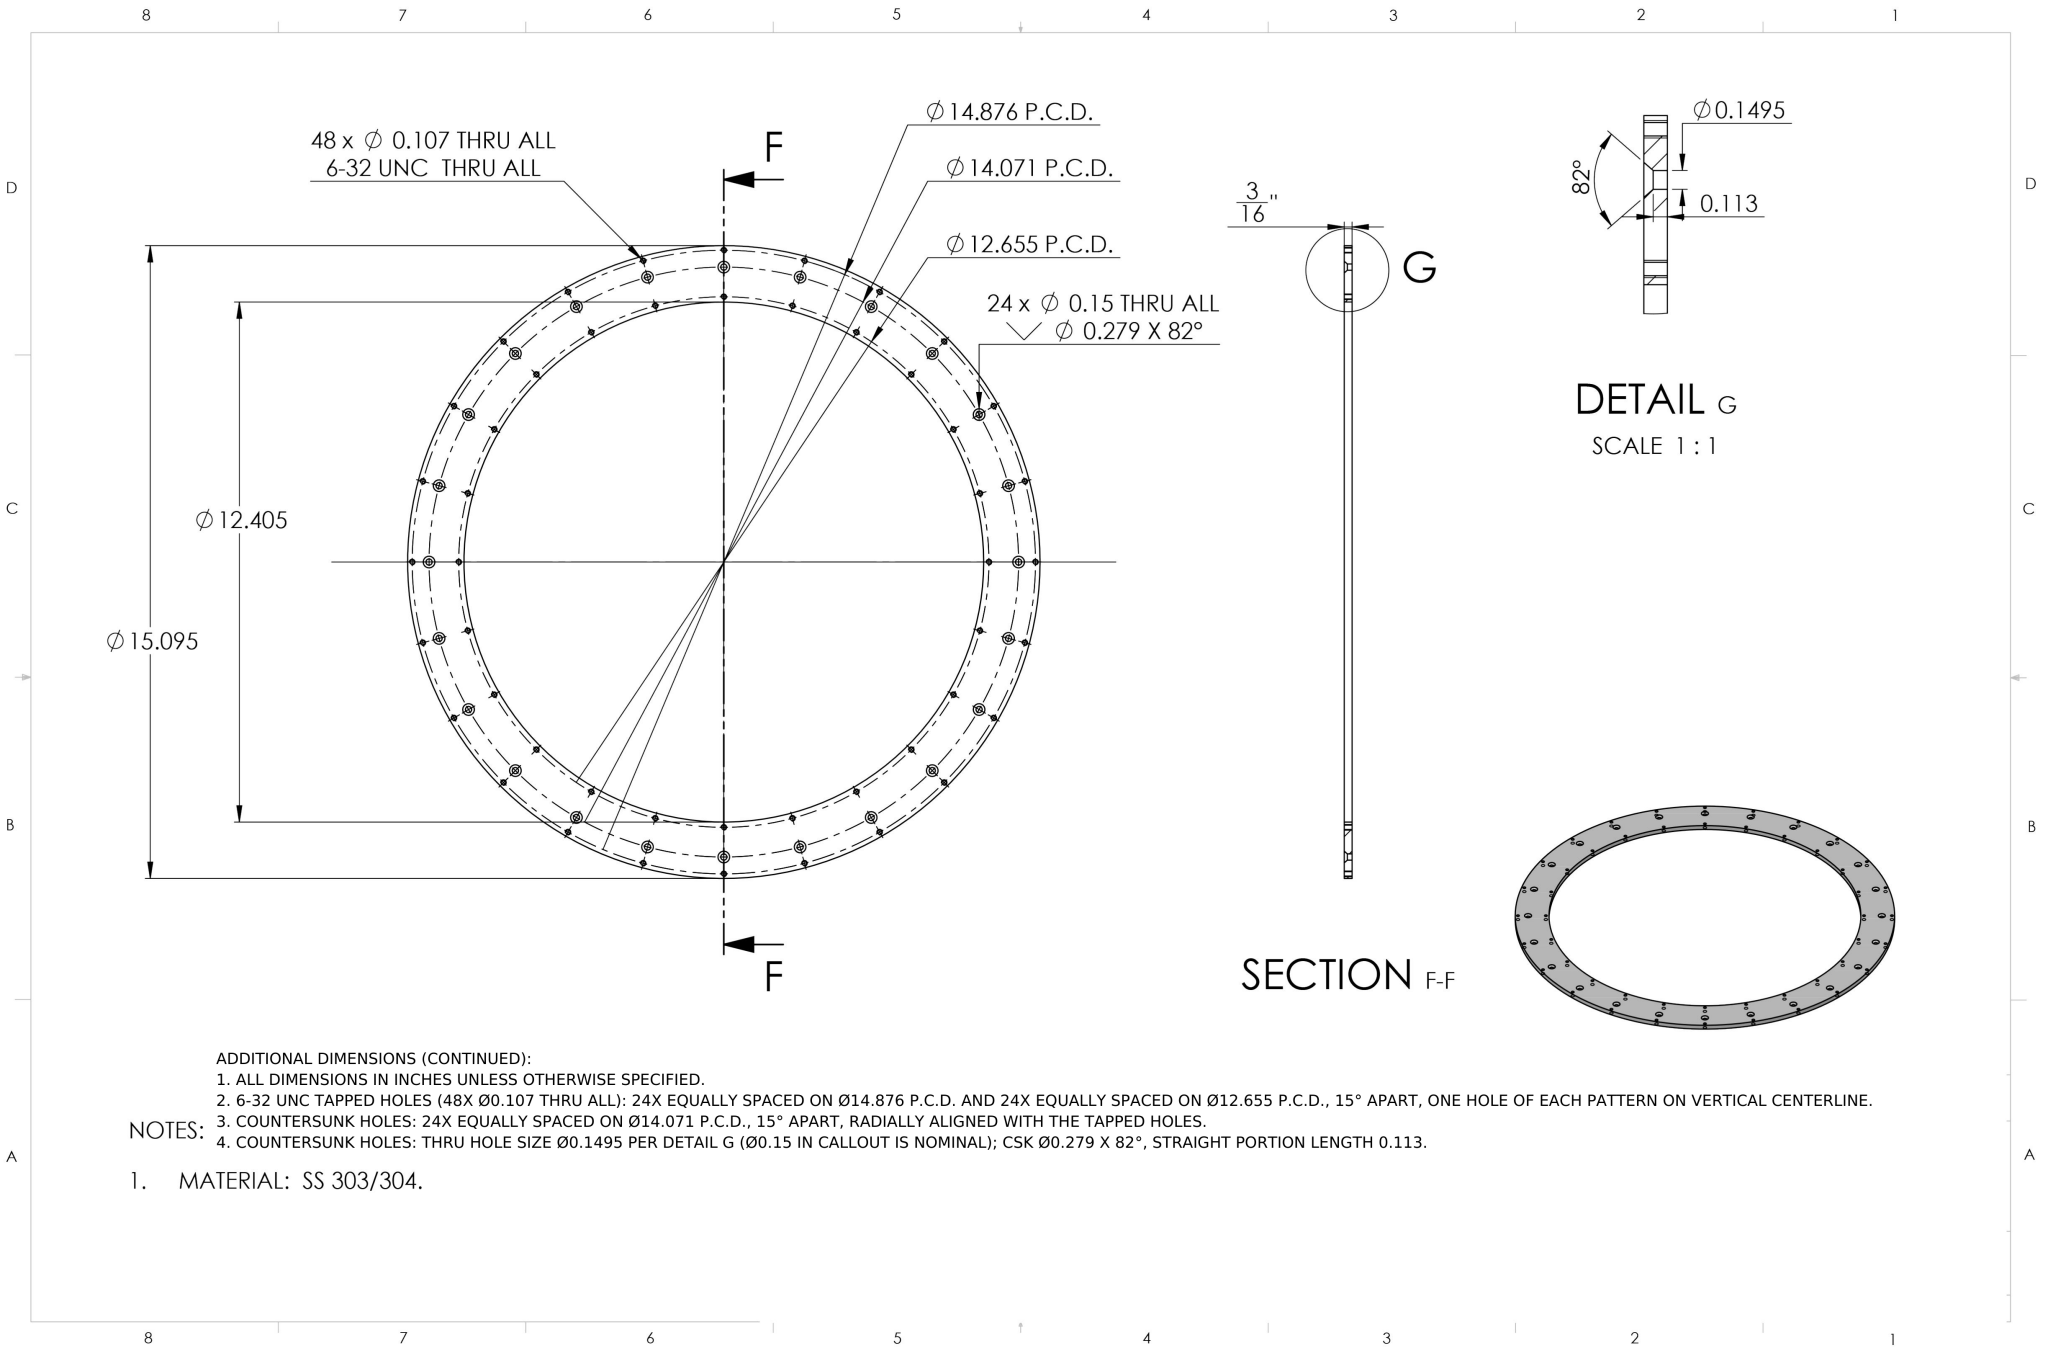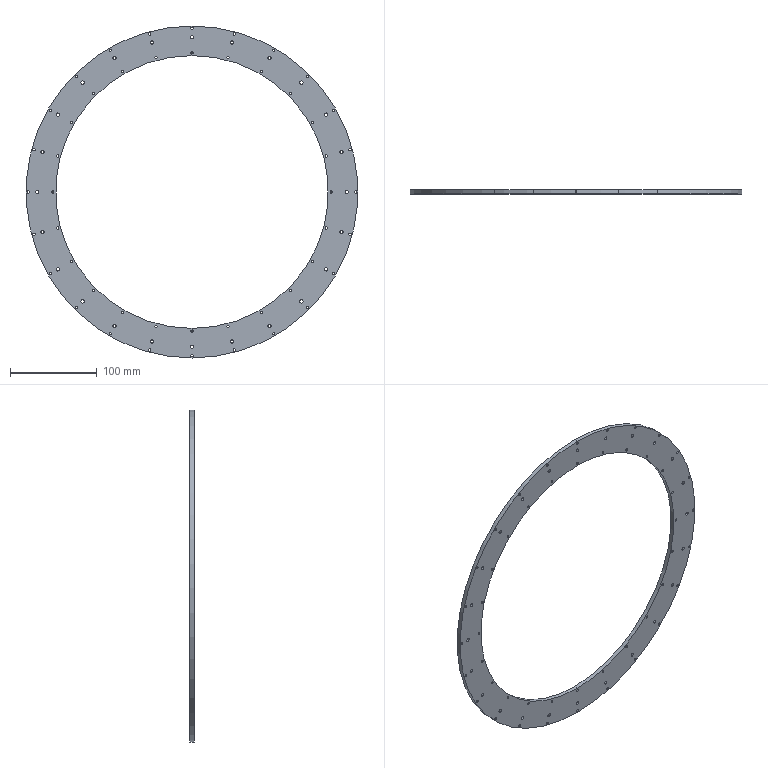Part | NX | drawing in inches | 1 solid | 198 faces | box 383.41 x 4.76 x 383.41 mm | volume 175334 mm3 | cylinder 148 | cone 48 | plane 2 | commonest cylinder face diameters 2.705 x96 3.797 x48 383.413 x2 315.087 x2